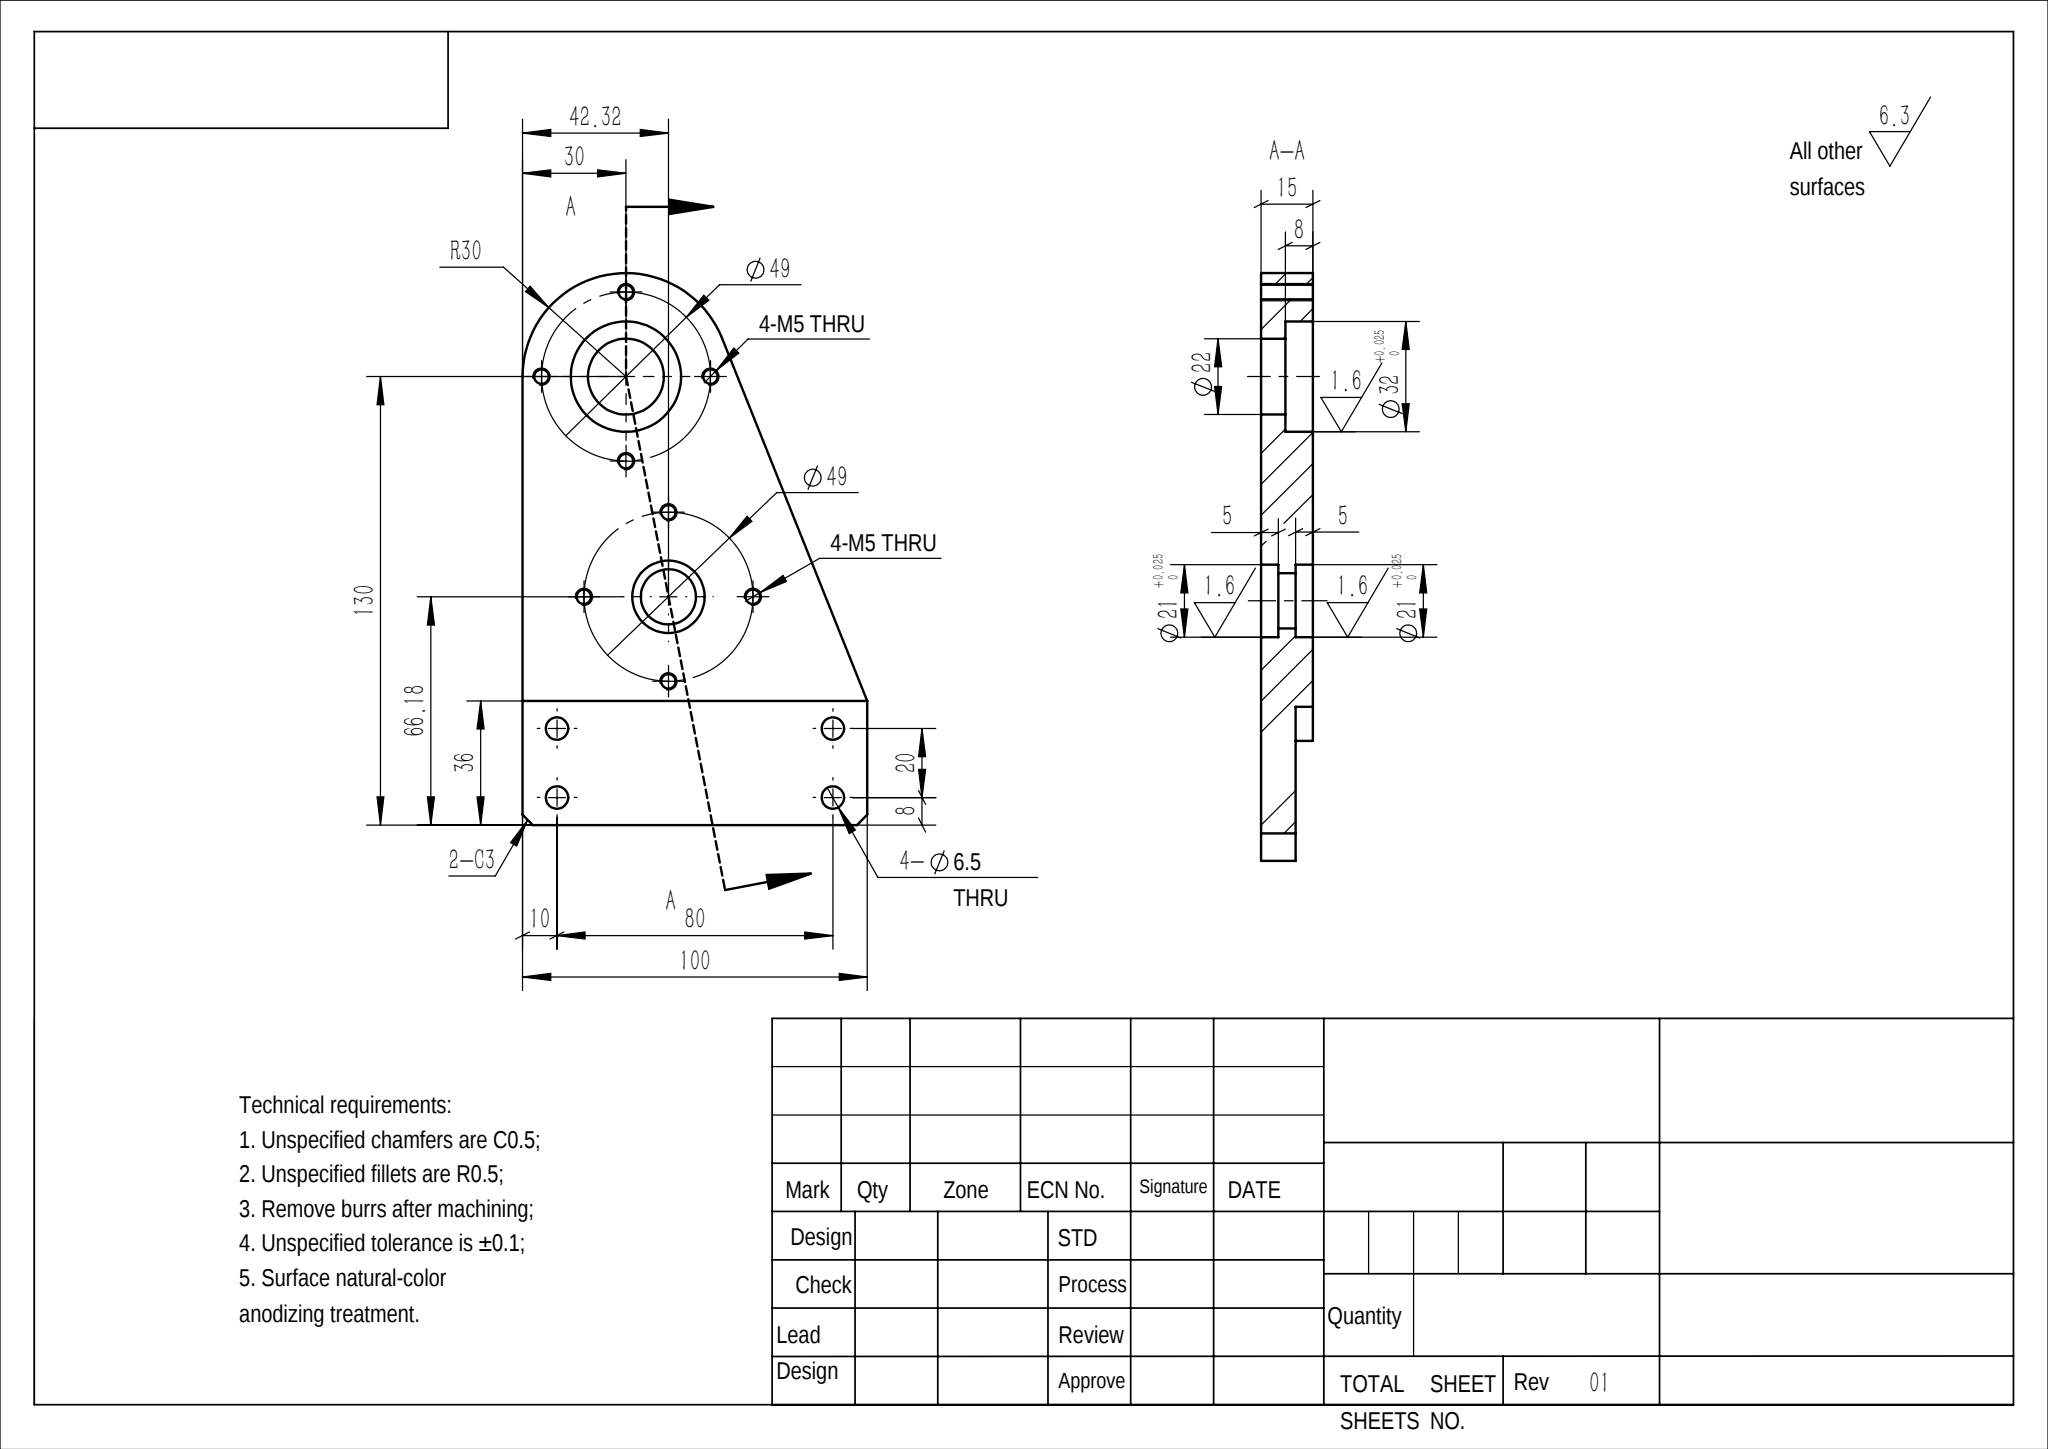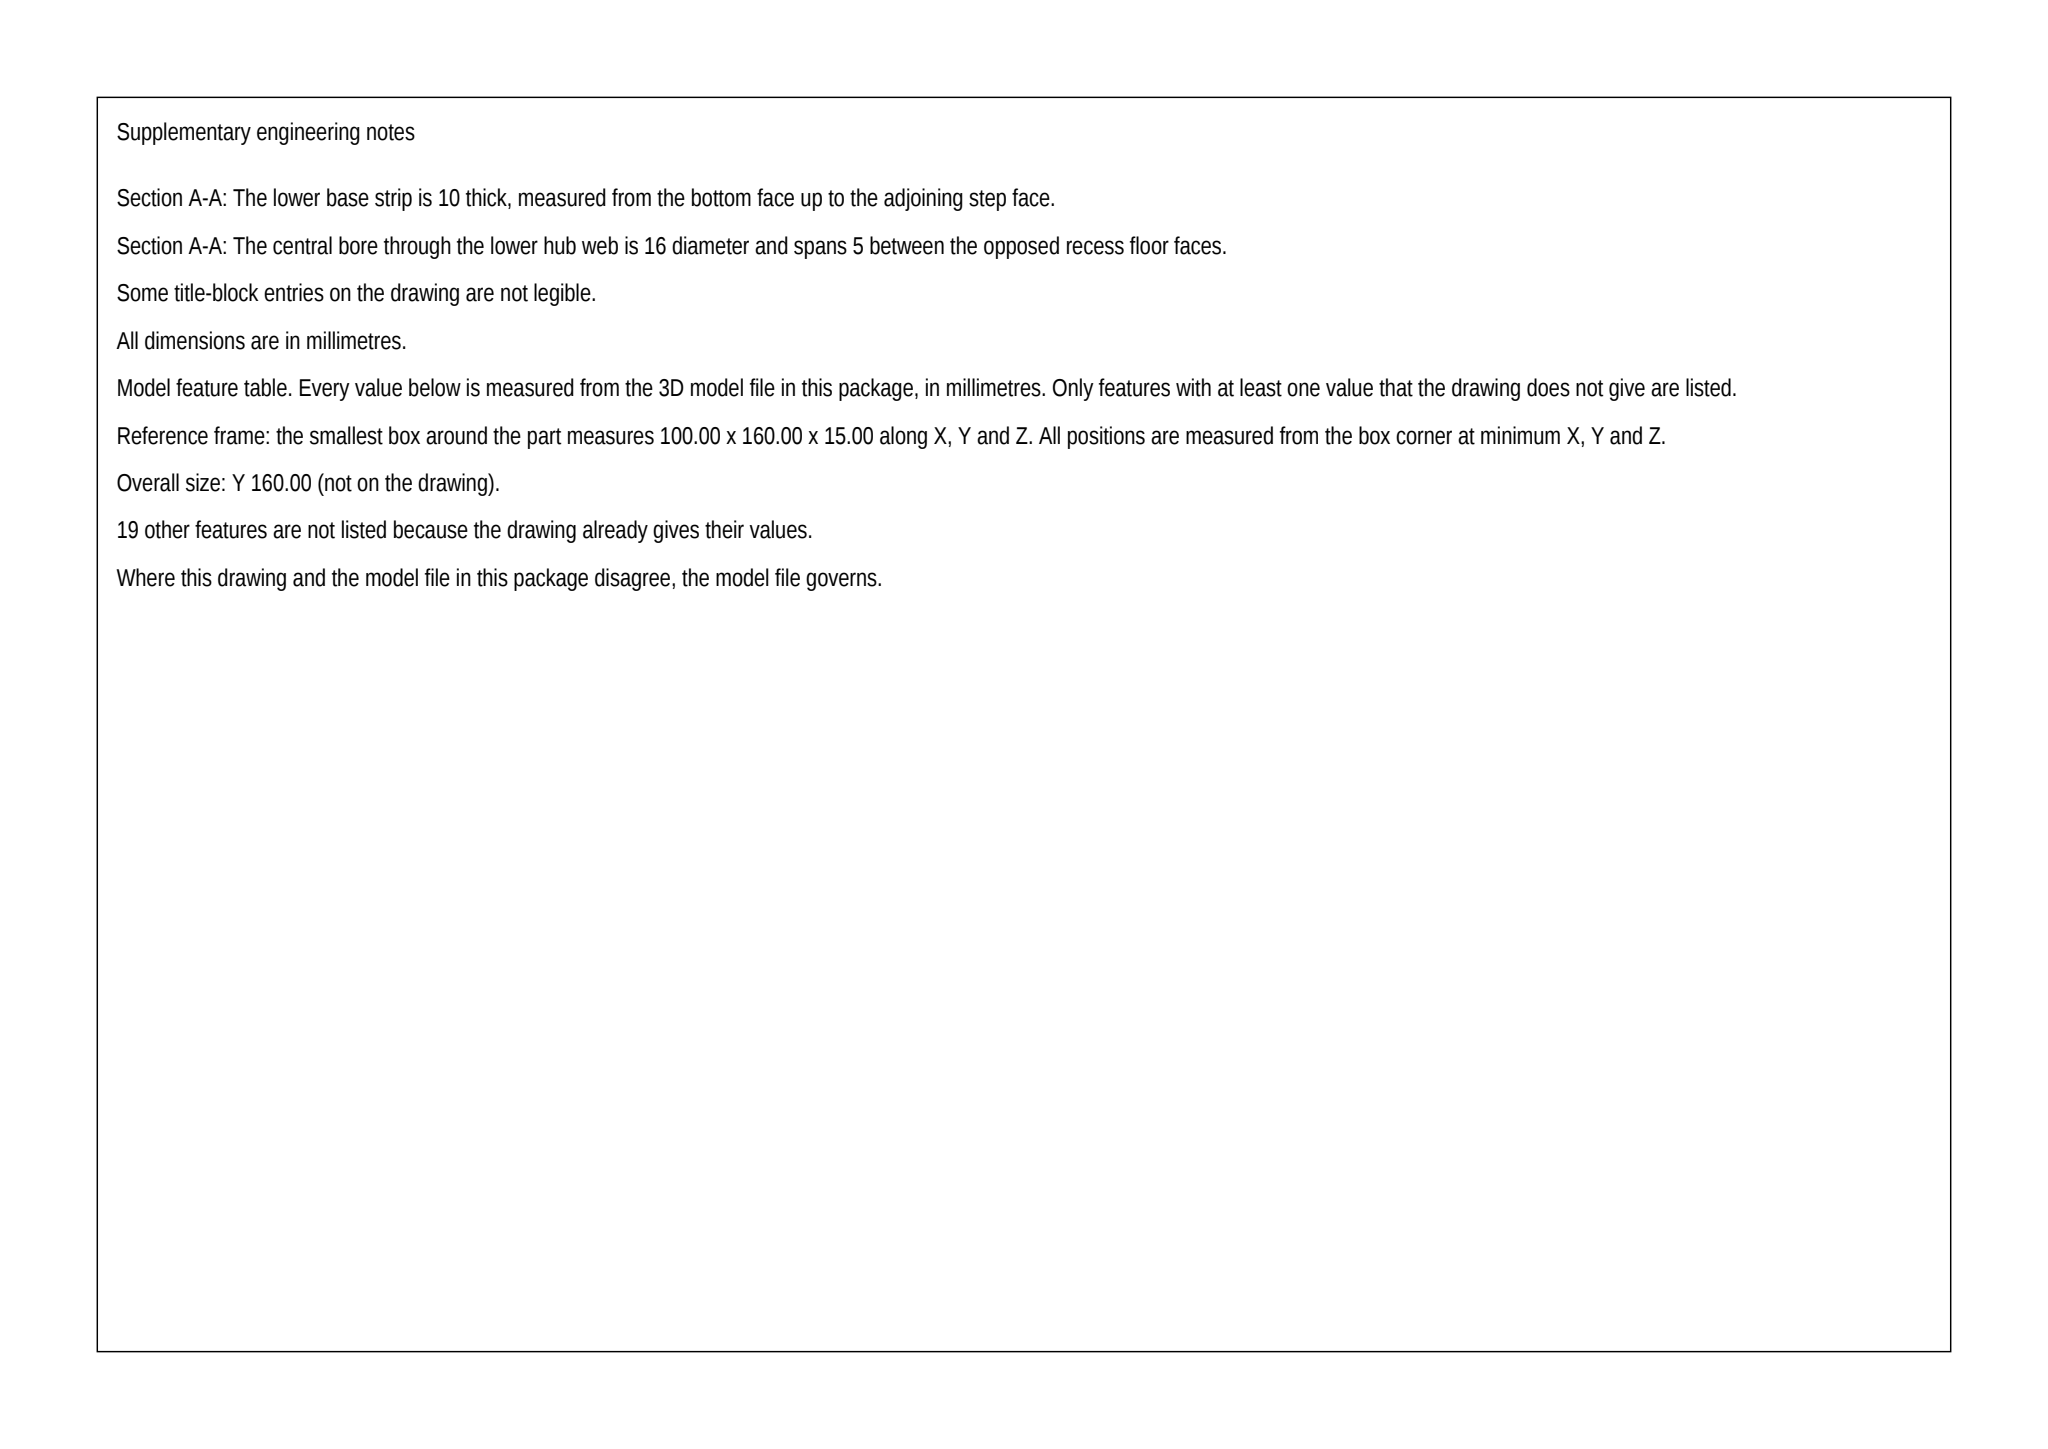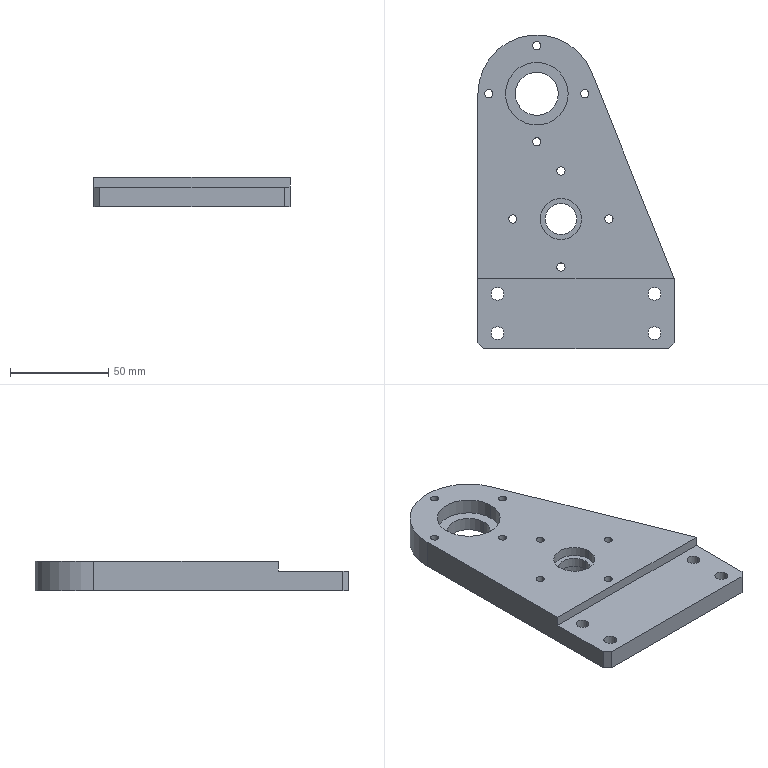Part | SolidWorks | mm | 1 solid | 48 faces | box 100 x 160 x 15 mm | volume 155130 mm3 | cylinder 35 | plane 13 | commonest cylinder face diameters 4.2 x16 6.5 x8 21 x4 32 x2 22 x2 16 x2 60 x1
build123d program:
from build123d import *

# Parameters (mm, degrees)
BOSS_EXTRUDE1_DEPTH = 15
SKETCH2_W           = 100
SKETCH2_H           = 36
CUT_EXTRUDE1_DEPTH  = 5
SKETCH3_R           = 3.25
CUT_EXTRUDE2_DEPTH  = 169.3
SKETCH4_R           = 11
SKETCH4_R_2         = 8
CUT_EXTRUDE3_DEPTH  = 169.3
SKETCH5_R           = 16
CUT_EXTRUDE4_DEPTH  = 8
SKETCH8_R           = 10.5
CUT_EXTRUDE5_DEPTH  = 5
CUT_EXTRUDE6_START  = -5
SKETCH9_R           = 10.5
CUT_EXTRUDE6_DEPTH  = 5
M5_TAPPED_HOLE1_D   = 4.2
CHAMFER1_SIZE       = 3


with BuildPart() as part:
    # Sketch1 → Boss-Extrude1 (new body)
    with BuildSketch(Plane.XY):
        with BuildLine():
            Line((-50, 0), (50, 0))
            Line((50, 0), (50, 36))
            Line((50, 36), (7.846, 141.162))
            ThreePointArc((7.846, 141.162), (-25.684, 159.457), (-50, 130))
            Line((-50, 130), (-50, 0))
        make_face()
    extrude(amount=BOSS_EXTRUDE1_DEPTH)

    # Sketch2 → Cut-Extrude1 (cut)
    with BuildSketch(Plane.XY.offset(15)):
        with Locations((0, 18)):
            Rectangle(SKETCH2_W, SKETCH2_H)
    extrude(amount=-CUT_EXTRUDE1_DEPTH, mode=Mode.SUBTRACT)

    # Sketch3 → Cut-Extrude2 (cut, through all)
    with BuildSketch(Plane(origin=(0, 0, 0), x_dir=(-1, 0, 0), z_dir=(0, 0, -1))):
        with Locations((-40, 28)):
            Circle(SKETCH3_R)
        with Locations(Location((40, 28, 0), (0, 0, 180))):
            Circle(SKETCH3_R)
        with Locations((-40, 8)):
            Circle(SKETCH3_R)
        with Locations(Location((40, 8, 0), (0, 0, 180))):
            Circle(SKETCH3_R)
    extrude(amount=-CUT_EXTRUDE2_DEPTH, mode=Mode.SUBTRACT)

    # Sketch4 → Cut-Extrude3 (cut, through all)
    with BuildSketch(Plane.XY.offset(15)):
        with Locations((-20, 130)):
            Circle(SKETCH4_R)
        with Locations((-7.685, 66.177)):
            Circle(SKETCH4_R_2)
    extrude(amount=-CUT_EXTRUDE3_DEPTH, mode=Mode.SUBTRACT)

    # Sketch5 → Cut-Extrude4 (cut)
    with BuildSketch(Plane.XY.offset(15)):
        with Locations((-20, 130)):
            Circle(SKETCH5_R)
    extrude(amount=-CUT_EXTRUDE4_DEPTH, mode=Mode.SUBTRACT)

    # Sketch8 → Cut-Extrude5 (cut)
    with BuildSketch(Plane.XY.offset(15)):
        with Locations((-7.685, 66.177)):
            Circle(SKETCH8_R)
    extrude(amount=-CUT_EXTRUDE5_DEPTH, mode=Mode.SUBTRACT)

    # Sketch9 → Cut-Extrude6 (cut)
    with BuildSketch(Plane(origin=(0, 0, 0), x_dir=(-1, 0, 0), z_dir=(0, 0, -1)).offset(CUT_EXTRUDE6_START)):
        with Locations(Location((7.685, 66.177, 0), (0, 0, 180))):
            Circle(SKETCH9_R)
    extrude(amount=CUT_EXTRUDE6_DEPTH, mode=Mode.SUBTRACT)

    # M5 Tapped Hole1 (through all)
    with Locations(Plane.XY.offset(15)):
        with Locations((-20, 154.5), (-20, 105.5), (-44.5, 130), (4.5, 130), (-7.685, 90.677), (-7.685, 41.677), (-32.185, 66.177), (16.815, 66.177)):
            Hole(M5_TAPPED_HOLE1_D / 2)

    # Chamfer1
    chamfer1_edges = [part.edges().sort_by_distance(p)[0] for p in [
        (50, 0, 5),
        (-50, 0, 5),
    ]]
    chamfer(chamfer1_edges, length=CHAMFER1_SIZE)


solid = part.part